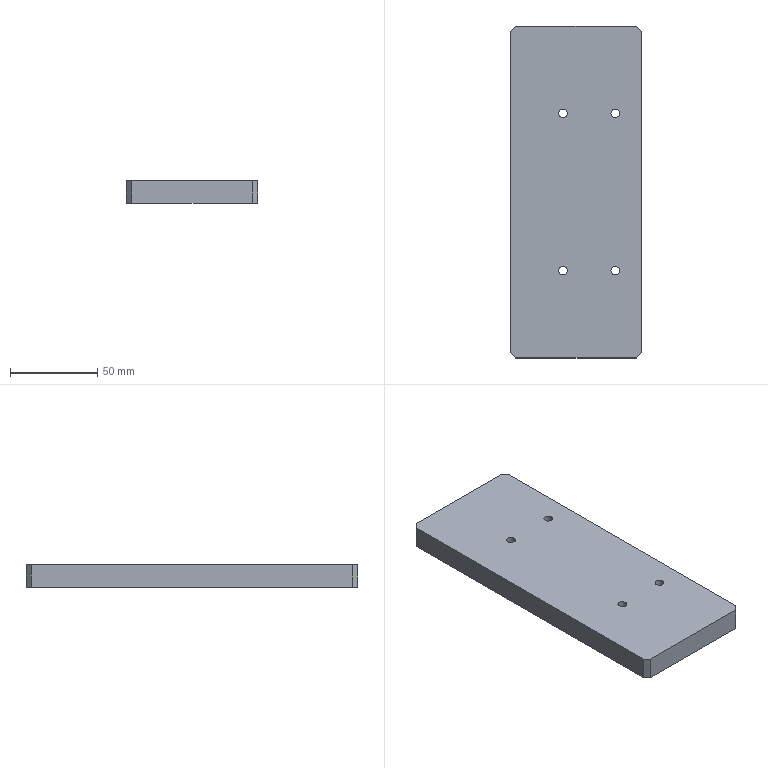Component | SolidWorks | STE21014.01-39-1 | 1 solid | 18 faces | box 75 x 190 x 13 mm | volume 183995 mm3 | plane 10 | cylinder 8 | commonest cylinder face diameters 5 x8 | material Q235
build123d program:
from build123d import *

# Parameters (mm, degrees)
SKETCH1_W           = 190
SKETCH1_H           = 75
BOSS_EXTRUDE1_DEPTH = 13
M6_TAPPED_HOLE1_D   = 5
CHAMFER1_SIZE       = 3


with BuildPart() as part:
    # Sketch1 → Boss-Extrude1 (new body)
    with BuildSketch(Plane(origin=(0, 0, 0), x_dir=(1, 0, 0), z_dir=(0, 1, 0))):
        Rectangle(SKETCH1_W, SKETCH1_H)
    extrude(amount=BOSS_EXTRUDE1_DEPTH)

    # M6 Tapped Hole1 (through all)
    with Locations(Plane(origin=(0, 13, 0), x_dir=(1, 0, 0), z_dir=(0, 1, 0))):
        with Locations((45, -7.5), (45, 22.5), (-45, -7.5), (-45, 22.5)):
            Hole(M6_TAPPED_HOLE1_D / 2)

    # Chamfer1
    chamfer1_edges = [part.edges().sort_by_distance(p)[0] for p in [
        (-95, 6.5, -37.5),
        (95, 6.5, -37.5),
        (95, 6.5, 37.5),
        (-95, 6.5, 37.5),
    ]]
    chamfer(chamfer1_edges, length=CHAMFER1_SIZE)


solid = part.part

# Placed as in the assembly
solid = solid.moved(Location((107.5, 80, -623), (90, -90, 0)))
STEP:
#1=COLOUR_RGB('',0.7922,0.8196,0.9333);
#2=FILL_AREA_STYLE_COLOUR('',#1);
#3=FILL_AREA_STYLE('',(#2));
#4=SURFACE_STYLE_FILL_AREA(#3);
#5=SURFACE_SIDE_STYLE('',(#4));
#6=SURFACE_STYLE_USAGE(.BOTH.,#5);
#7=PRESENTATION_STYLE_ASSIGNMENT((#6));
#8=CARTESIAN_POINT('',(4.035,4.921,-24.016));
#9=VERTEX_POINT('',#8);
#10=CARTESIAN_POINT('',(3.839,4.921,-24.016));
#11=VERTEX_POINT('',#10);
#12=CARTESIAN_POINT('',(3.937,4.921,-24.016));
#13=DIRECTION('',(-0.,-0.,-1.));
#14=DIRECTION('',(-1.,0.,0.));
#15=AXIS2_PLACEMENT_3D('',#12,#13,#14);
#16=CIRCLE('',#15,0.09843);
#17=EDGE_CURVE('',#9,#11,#16,.T.);
#18=ORIENTED_EDGE('',*,*,#17,.F.);
#19=CARTESIAN_POINT('',(4.035,4.921,-24.528));
#20=VERTEX_POINT('',#19);
#21=CARTESIAN_POINT('',(4.035,4.921,-24.528));
#22=DIRECTION('',(-0.,-0.,-1.));
#23=VECTOR('',#22,39.37);
#24=LINE('',#21,#23);
#25=EDGE_CURVE('',#9,#20,#24,.T.);
#26=ORIENTED_EDGE('',*,*,#25,.T.);
#27=CARTESIAN_POINT('',(3.839,4.921,-24.528));
#28=VERTEX_POINT('',#27);
#29=CARTESIAN_POINT('',(3.937,4.921,-24.528));
#30=DIRECTION('',(-0.,-0.,-1.));
#31=DIRECTION('',(-1.,0.,0.));
#32=AXIS2_PLACEMENT_3D('',#29,#30,#31);
#33=CIRCLE('',#32,0.09843);
#34=EDGE_CURVE('',#20,#28,#33,.T.);
#35=ORIENTED_EDGE('',*,*,#34,.T.);
#36=CARTESIAN_POINT('',(3.839,4.921,-24.528));
#37=DIRECTION('',(-0.,-0.,-1.));
#38=VECTOR('',#37,39.37);
#39=LINE('',#36,#38);
#40=EDGE_CURVE('',#11,#28,#39,.T.);
#41=ORIENTED_EDGE('',*,*,#40,.F.);
#42=EDGE_LOOP('',(#18,#26,#35,#41));
#43=FACE_OUTER_BOUND('',#42,.T.);
#44=CARTESIAN_POINT('',(3.937,4.921,-24.528));
#45=DIRECTION('',(-0.,-0.,-1.));
#46=DIRECTION('',(-1.,0.,0.));
#47=AXIS2_PLACEMENT_3D('',#44,#45,#46);
#48=CYLINDRICAL_SURFACE('',#47,0.09843);
#49=ADVANCED_FACE('',(#43),#48,.F.);
#50=CARTESIAN_POINT('',(5.217,4.921,-24.016));
#51=VERTEX_POINT('',#50);
#52=CARTESIAN_POINT('',(5.02,4.921,-24.016));
#53=VERTEX_POINT('',#52);
#54=CARTESIAN_POINT('',(5.118,4.921,-24.016));
#55=DIRECTION('',(-0.,-0.,-1.));
#56=DIRECTION('',(-1.,0.,0.));
#57=AXIS2_PLACEMENT_3D('',#54,#55,#56);
#58=CIRCLE('',#57,0.09843);
#59=EDGE_CURVE('',#51,#53,#58,.T.);
#60=ORIENTED_EDGE('',*,*,#59,.F.);
#61=CARTESIAN_POINT('',(5.217,4.921,-24.528));
#62=VERTEX_POINT('',#61);
#63=CARTESIAN_POINT('',(5.217,4.921,-24.528));
#64=DIRECTION('',(-0.,-0.,-1.));
#65=VECTOR('',#64,39.37);
#66=LINE('',#63,#65);
#67=EDGE_CURVE('',#51,#62,#66,.T.);
#68=ORIENTED_EDGE('',*,*,#67,.T.);
#69=CARTESIAN_POINT('',(5.02,4.921,-24.528));
#70=VERTEX_POINT('',#69);
#71=CARTESIAN_POINT('',(5.118,4.921,-24.528));
#72=DIRECTION('',(-0.,-0.,-1.));
#73=DIRECTION('',(-1.,0.,0.));
#74=AXIS2_PLACEMENT_3D('',#71,#72,#73);
#75=CIRCLE('',#74,0.09843);
#76=EDGE_CURVE('',#62,#70,#75,.T.);
#77=ORIENTED_EDGE('',*,*,#76,.T.);
#78=CARTESIAN_POINT('',(5.02,4.921,-24.528));
#79=DIRECTION('',(-0.,-0.,-1.));
#80=VECTOR('',#79,39.37);
#81=LINE('',#78,#80);
#82=EDGE_CURVE('',#53,#70,#81,.T.);
#83=ORIENTED_EDGE('',*,*,#82,.F.);
#84=EDGE_LOOP('',(#60,#68,#77,#83));
#85=FACE_OUTER_BOUND('',#84,.T.);
#86=CARTESIAN_POINT('',(5.118,4.921,-24.528));
#87=DIRECTION('',(-0.,-0.,-1.));
#88=DIRECTION('',(-1.,0.,0.));
#89=AXIS2_PLACEMENT_3D('',#86,#87,#88);
#90=CYLINDRICAL_SURFACE('',#89,0.09843);
#91=ADVANCED_FACE('',(#85),#90,.F.);
#92=CARTESIAN_POINT('',(4.035,1.378,-24.016));
#93=VERTEX_POINT('',#92);
#94=CARTESIAN_POINT('',(3.839,1.378,-24.016));
#95=VERTEX_POINT('',#94);
#96=CARTESIAN_POINT('',(3.937,1.378,-24.016));
#97=DIRECTION('',(-0.,-0.,-1.));
#98=DIRECTION('',(-1.,0.,0.));
#99=AXIS2_PLACEMENT_3D('',#96,#97,#98);
#100=CIRCLE('',#99,0.09843);
#101=EDGE_CURVE('',#93,#95,#100,.T.);
#102=ORIENTED_EDGE('',*,*,#101,.F.);
#103=CARTESIAN_POINT('',(4.035,1.378,-24.528));
#104=VERTEX_POINT('',#103);
#105=CARTESIAN_POINT('',(4.035,1.378,-24.528));
#106=DIRECTION('',(-0.,-0.,-1.));
#107=VECTOR('',#106,39.37);
#108=LINE('',#105,#107);
#109=EDGE_CURVE('',#93,#104,#108,.T.);
#110=ORIENTED_EDGE('',*,*,#109,.T.);
#111=CARTESIAN_POINT('',(3.839,1.378,-24.528));
#112=VERTEX_POINT('',#111);
#113=CARTESIAN_POINT('',(3.937,1.378,-24.528));
#114=DIRECTION('',(-0.,-0.,-1.));
#115=DIRECTION('',(-1.,0.,0.));
#116=AXIS2_PLACEMENT_3D('',#113,#114,#115);
#117=CIRCLE('',#116,0.09843);
#118=EDGE_CURVE('',#104,#112,#117,.T.);
#119=ORIENTED_EDGE('',*,*,#118,.T.);
#120=CARTESIAN_POINT('',(3.839,1.378,-24.528));
#121=DIRECTION('',(-0.,-0.,-1.));
#122=VECTOR('',#121,39.37);
#123=LINE('',#120,#122);
#124=EDGE_CURVE('',#95,#112,#123,.T.);
#125=ORIENTED_EDGE('',*,*,#124,.F.);
#126=EDGE_LOOP('',(#102,#110,#119,#125));
#127=FACE_OUTER_BOUND('',#126,.T.);
#128=CARTESIAN_POINT('',(3.937,1.378,-24.528));
#129=DIRECTION('',(-0.,-0.,-1.));
#130=DIRECTION('',(-1.,0.,0.));
#131=AXIS2_PLACEMENT_3D('',#128,#129,#130);
#132=CYLINDRICAL_SURFACE('',#131,0.09843);
#133=ADVANCED_FACE('',(#127),#132,.F.);
#134=CARTESIAN_POINT('',(5.217,1.378,-24.016));
#135=VERTEX_POINT('',#134);
#136=CARTESIAN_POINT('',(5.02,1.378,-24.016));
#137=VERTEX_POINT('',#136);
#138=CARTESIAN_POINT('',(5.118,1.378,-24.016));
#139=DIRECTION('',(-0.,-0.,-1.));
#140=DIRECTION('',(-1.,0.,0.));
#141=AXIS2_PLACEMENT_3D('',#138,#139,#140);
#142=CIRCLE('',#141,0.09843);
#143=EDGE_CURVE('',#135,#137,#142,.T.);
#144=ORIENTED_EDGE('',*,*,#143,.F.);
#145=CARTESIAN_POINT('',(5.217,1.378,-24.528));
#146=VERTEX_POINT('',#145);
#147=CARTESIAN_POINT('',(5.217,1.378,-24.528));
#148=DIRECTION('',(-0.,-0.,-1.));
#149=VECTOR('',#148,39.37);
#150=LINE('',#147,#149);
#151=EDGE_CURVE('',#135,#146,#150,.T.);
#152=ORIENTED_EDGE('',*,*,#151,.T.);
#153=CARTESIAN_POINT('',(5.02,1.378,-24.528));
#154=VERTEX_POINT('',#153);
#155=CARTESIAN_POINT('',(5.118,1.378,-24.528));
#156=DIRECTION('',(-0.,-0.,-1.));
#157=DIRECTION('',(-1.,0.,0.));
#158=AXIS2_PLACEMENT_3D('',#155,#156,#157);
#159=CIRCLE('',#158,0.09843);
#160=EDGE_CURVE('',#146,#154,#159,.T.);
#161=ORIENTED_EDGE('',*,*,#160,.T.);
#162=CARTESIAN_POINT('',(5.02,1.378,-24.528));
#163=DIRECTION('',(-0.,-0.,-1.));
#164=VECTOR('',#163,39.37);
#165=LINE('',#162,#164);
#166=EDGE_CURVE('',#137,#154,#165,.T.);
#167=ORIENTED_EDGE('',*,*,#166,.F.);
#168=EDGE_LOOP('',(#144,#152,#161,#167));
#169=FACE_OUTER_BOUND('',#168,.T.);
#170=CARTESIAN_POINT('',(5.118,1.378,-24.528));
#171=DIRECTION('',(-0.,-0.,-1.));
#172=DIRECTION('',(-1.,0.,0.));
#173=AXIS2_PLACEMENT_3D('',#170,#171,#172);
#174=CYLINDRICAL_SURFACE('',#173,0.09843);
#175=ADVANCED_FACE('',(#169),#174,.F.);
#176=CARTESIAN_POINT('',(5.591,-0.5906,-24.528));
#177=VERTEX_POINT('',#176);
#178=CARTESIAN_POINT('',(2.874,-0.5906,-24.528));
#179=VERTEX_POINT('',#178);
#180=CARTESIAN_POINT('',(2.756,-0.5906,-24.528));
#181=DIRECTION('',(-1.,-0.,0.));
#182=VECTOR('',#181,39.37);
#183=LINE('',#180,#182);
#184=EDGE_CURVE('',#177,#179,#183,.T.);
#185=ORIENTED_EDGE('',*,*,#184,.F.);
#186=CARTESIAN_POINT('',(5.591,-0.5906,-24.016));
#187=VERTEX_POINT('',#186);
#188=CARTESIAN_POINT('',(5.591,-0.5906,-24.528));
#189=DIRECTION('',(0.,0.,1.));
#190=VECTOR('',#189,39.37);
#191=LINE('',#188,#190);
#192=EDGE_CURVE('',#177,#187,#191,.T.);
#193=ORIENTED_EDGE('',*,*,#192,.T.);
#194=CARTESIAN_POINT('',(2.874,-0.5906,-24.016));
#195=VERTEX_POINT('',#194);
#196=CARTESIAN_POINT('',(2.756,-0.5906,-24.016));
#197=DIRECTION('',(-1.,-0.,0.));
#198=VECTOR('',#197,39.37);
#199=LINE('',#196,#198);
#200=EDGE_CURVE('',#187,#195,#199,.T.);
#201=ORIENTED_EDGE('',*,*,#200,.T.);
#202=CARTESIAN_POINT('',(2.874,-0.5906,-24.528));
#203=DIRECTION('',(-0.,-0.,-1.));
#204=VECTOR('',#203,39.37);
#205=LINE('',#202,#204);
#206=EDGE_CURVE('',#195,#179,#205,.T.);
#207=ORIENTED_EDGE('',*,*,#206,.T.);
#208=EDGE_LOOP('',(#185,#193,#201,#207));
#209=FACE_OUTER_BOUND('',#208,.T.);
#210=CARTESIAN_POINT('',(2.756,-0.5906,-24.528));
#211=DIRECTION('',(-0.,1.,-0.));
#212=DIRECTION('',(1.,0.,-0.));
#213=AXIS2_PLACEMENT_3D('',#210,#211,#212);
#214=PLANE('',#213);
#215=ADVANCED_FACE('',(#209),#214,.F.);
#216=CARTESIAN_POINT('',(2.756,-0.4724,-24.016));
#217=VERTEX_POINT('',#216);
#218=CARTESIAN_POINT('',(2.756,6.772,-24.016));
#219=VERTEX_POINT('',#218);
#220=CARTESIAN_POINT('',(2.756,6.89,-24.016));
#221=DIRECTION('',(0.,1.,-0.));
#222=VECTOR('',#221,39.37);
#223=LINE('',#220,#222);
#224=EDGE_CURVE('',#217,#219,#223,.T.);
#225=ORIENTED_EDGE('',*,*,#224,.T.);
#226=CARTESIAN_POINT('',(2.756,6.772,-24.528));
#227=VERTEX_POINT('',#226);
#228=CARTESIAN_POINT('',(2.756,6.772,-24.528));
#229=DIRECTION('',(-0.,-0.,-1.));
#230=VECTOR('',#229,39.37);
#231=LINE('',#228,#230);
#232=EDGE_CURVE('',#219,#227,#231,.T.);
#233=ORIENTED_EDGE('',*,*,#232,.T.);
#234=CARTESIAN_POINT('',(2.756,-0.4724,-24.528));
#235=VERTEX_POINT('',#234);
#236=CARTESIAN_POINT('',(2.756,6.89,-24.528));
#237=DIRECTION('',(0.,1.,-0.));
#238=VECTOR('',#237,39.37);
#239=LINE('',#236,#238);
#240=EDGE_CURVE('',#235,#227,#239,.T.);
#241=ORIENTED_EDGE('',*,*,#240,.F.);
#242=CARTESIAN_POINT('',(2.756,-0.4724,-24.528));
#243=DIRECTION('',(0.,0.,1.));
#244=VECTOR('',#243,39.37);
#245=LINE('',#242,#244);
#246=EDGE_CURVE('',#235,#217,#245,.T.);
#247=ORIENTED_EDGE('',*,*,#246,.T.);
#248=EDGE_LOOP('',(#225,#233,#241,#247));
#249=FACE_OUTER_BOUND('',#248,.T.);
#250=CARTESIAN_POINT('',(2.756,6.89,-24.528));
#251=DIRECTION('',(1.,-0.,-0.));
#252=DIRECTION('',(-0.,-1.,0.));
#253=AXIS2_PLACEMENT_3D('',#250,#251,#252);
#254=PLANE('',#253);
#255=ADVANCED_FACE('',(#249),#254,.F.);
#256=CARTESIAN_POINT('',(2.874,6.89,-24.528));
#257=VERTEX_POINT('',#256);
#258=CARTESIAN_POINT('',(5.591,6.89,-24.528));
#259=VERTEX_POINT('',#258);
#260=CARTESIAN_POINT('',(2.756,6.89,-24.528));
#261=DIRECTION('',(1.,0.,-0.));
#262=VECTOR('',#261,39.37);
#263=LINE('',#260,#262);
#264=EDGE_CURVE('',#257,#259,#263,.T.);
#265=ORIENTED_EDGE('',*,*,#264,.F.);
#266=CARTESIAN_POINT('',(2.874,6.89,-24.016));
#267=VERTEX_POINT('',#266);
#268=CARTESIAN_POINT('',(2.874,6.89,-24.528));
#269=DIRECTION('',(0.,0.,1.));
#270=VECTOR('',#269,39.37);
#271=LINE('',#268,#270);
#272=EDGE_CURVE('',#257,#267,#271,.T.);
#273=ORIENTED_EDGE('',*,*,#272,.T.);
#274=CARTESIAN_POINT('',(5.591,6.89,-24.016));
#275=VERTEX_POINT('',#274);
#276=CARTESIAN_POINT('',(2.756,6.89,-24.016));
#277=DIRECTION('',(1.,0.,-0.));
#278=VECTOR('',#277,39.37);
#279=LINE('',#276,#278);
#280=EDGE_CURVE('',#267,#275,#279,.T.);
#281=ORIENTED_EDGE('',*,*,#280,.T.);
#282=CARTESIAN_POINT('',(5.591,6.89,-24.528));
#283=DIRECTION('',(-0.,-0.,-1.));
#284=VECTOR('',#283,39.37);
#285=LINE('',#282,#284);
#286=EDGE_CURVE('',#275,#259,#285,.T.);
#287=ORIENTED_EDGE('',*,*,#286,.T.);
#288=EDGE_LOOP('',(#265,#273,#281,#287));
#289=FACE_OUTER_BOUND('',#288,.T.);
#290=CARTESIAN_POINT('',(2.756,6.89,-24.528));
#291=DIRECTION('',(0.,-1.,0.));
#292=DIRECTION('',(-1.,-0.,0.));
#293=AXIS2_PLACEMENT_3D('',#290,#291,#292);
#294=PLANE('',#293);
#295=ADVANCED_FACE('',(#289),#294,.F.);
#296=CARTESIAN_POINT('',(5.709,6.772,-24.528));
#297=VERTEX_POINT('',#296);
#298=CARTESIAN_POINT('',(5.709,-0.4724,-24.528));
#299=VERTEX_POINT('',#298);
#300=CARTESIAN_POINT('',(5.709,6.89,-24.528));
#301=DIRECTION('',(-0.,-1.,0.));
#302=VECTOR('',#301,39.37);
#303=LINE('',#300,#302);
#304=EDGE_CURVE('',#297,#299,#303,.T.);
#305=ORIENTED_EDGE('',*,*,#304,.F.);
#306=CARTESIAN_POINT('',(5.709,6.772,-24.016));
#307=VERTEX_POINT('',#306);
#308=CARTESIAN_POINT('',(5.709,6.772,-24.528));
#309=DIRECTION('',(0.,0.,1.));
#310=VECTOR('',#309,39.37);
#311=LINE('',#308,#310);
#312=EDGE_CURVE('',#297,#307,#311,.T.);
#313=ORIENTED_EDGE('',*,*,#312,.T.);
#314=CARTESIAN_POINT('',(5.709,-0.4724,-24.016));
#315=VERTEX_POINT('',#314);
#316=CARTESIAN_POINT('',(5.709,6.89,-24.016));
#317=DIRECTION('',(-0.,-1.,0.));
#318=VECTOR('',#317,39.37);
#319=LINE('',#316,#318);
#320=EDGE_CURVE('',#307,#315,#319,.T.);
#321=ORIENTED_EDGE('',*,*,#320,.T.);
#322=CARTESIAN_POINT('',(5.709,-0.4724,-24.528));
#323=DIRECTION('',(-0.,-0.,-1.));
#324=VECTOR('',#323,39.37);
#325=LINE('',#322,#324);
#326=EDGE_CURVE('',#315,#299,#325,.T.);
#327=ORIENTED_EDGE('',*,*,#326,.T.);
#328=EDGE_LOOP('',(#305,#313,#321,#327));
#329=FACE_OUTER_BOUND('',#328,.T.);
#330=CARTESIAN_POINT('',(5.709,6.89,-24.528));
#331=DIRECTION('',(-1.,0.,0.));
#332=DIRECTION('',(0.,1.,-0.));
#333=AXIS2_PLACEMENT_3D('',#330,#331,#332);
#334=PLANE('',#333);
#335=ADVANCED_FACE('',(#329),#334,.F.);
#336=CARTESIAN_POINT('',(3.937,4.921,-24.528));
#337=DIRECTION('',(-0.,-0.,-1.));
#338=DIRECTION('',(-1.,0.,0.));
#339=AXIS2_PLACEMENT_3D('',#336,#337,#338);
#340=CIRCLE('',#339,0.09843);
#341=EDGE_CURVE('',#28,#20,#340,.T.);
#342=ORIENTED_EDGE('',*,*,#341,.F.);
#343=ORIENTED_EDGE('',*,*,#34,.F.);
#344=EDGE_LOOP('',(#342,#343));
#345=FACE_BOUND('',#344,.T.);
#346=CARTESIAN_POINT('',(5.118,4.921,-24.528));
#347=DIRECTION('',(-0.,-0.,-1.));
#348=DIRECTION('',(-1.,0.,0.));
#349=AXIS2_PLACEMENT_3D('',#346,#347,#348);
#350=CIRCLE('',#349,0.09843);
#351=EDGE_CURVE('',#70,#62,#350,.T.);
#352=ORIENTED_EDGE('',*,*,#351,.F.);
#353=ORIENTED_EDGE('',*,*,#76,.F.);
#354=EDGE_LOOP('',(#352,#353));
#355=FACE_BOUND('',#354,.T.);
#356=CARTESIAN_POINT('',(3.937,1.378,-24.528));
#357=DIRECTION('',(-0.,-0.,-1.));
#358=DIRECTION('',(-1.,0.,0.));
#359=AXIS2_PLACEMENT_3D('',#356,#357,#358);
#360=CIRCLE('',#359,0.09843);
#361=EDGE_CURVE('',#112,#104,#360,.T.);
#362=ORIENTED_EDGE('',*,*,#361,.F.);
#363=ORIENTED_EDGE('',*,*,#118,.F.);
#364=EDGE_LOOP('',(#362,#363));
#365=FACE_BOUND('',#364,.T.);
#366=CARTESIAN_POINT('',(5.118,1.378,-24.528));
#367=DIRECTION('',(-0.,-0.,-1.));
#368=DIRECTION('',(-1.,0.,0.));
#369=AXIS2_PLACEMENT_3D('',#366,#367,#368);
#370=CIRCLE('',#369,0.09843);
#371=EDGE_CURVE('',#154,#146,#370,.T.);
#372=ORIENTED_EDGE('',*,*,#371,.F.);
#373=ORIENTED_EDGE('',*,*,#160,.F.);
#374=EDGE_LOOP('',(#372,#373));
#375=FACE_BOUND('',#374,.T.);
#376=ORIENTED_EDGE('',*,*,#240,.T.);
#377=CARTESIAN_POINT('',(1.683,5.699,-24.528));
#378=DIRECTION('',(0.7071,0.7071,-0.));
#379=VECTOR('',#378,39.37);
#380=LINE('',#377,#379);
#381=EDGE_CURVE('',#227,#257,#380,.T.);
#382=ORIENTED_EDGE('',*,*,#381,.T.);
#383=ORIENTED_EDGE('',*,*,#264,.T.);
#384=CARTESIAN_POINT('',(6.781,5.699,-24.528));
#385=DIRECTION('',(0.7071,-0.7071,0.));
#386=VECTOR('',#385,39.37);
#387=LINE('',#384,#386);
#388=EDGE_CURVE('',#259,#297,#387,.T.);
#389=ORIENTED_EDGE('',*,*,#388,.T.);
#390=ORIENTED_EDGE('',*,*,#304,.T.);
#391=CARTESIAN_POINT('',(6.781,0.6004,-24.528));
#392=DIRECTION('',(-0.7071,-0.7071,0.));
#393=VECTOR('',#392,39.37);
#394=LINE('',#391,#393);
#395=EDGE_CURVE('',#299,#177,#394,.T.);
#396=ORIENTED_EDGE('',*,*,#395,.T.);
#397=ORIENTED_EDGE('',*,*,#184,.T.);
#398=CARTESIAN_POINT('',(1.683,0.6004,-24.528));
#399=DIRECTION('',(-0.7071,0.7071,-0.));
#400=VECTOR('',#399,39.37);
#401=LINE('',#398,#400);
#402=EDGE_CURVE('',#179,#235,#401,.T.);
#403=ORIENTED_EDGE('',*,*,#402,.T.);
#404=EDGE_LOOP('',(#376,#382,#383,#389,#390,#396,#397,#403));
#405=FACE_OUTER_BOUND('',#404,.T.);
#406=CARTESIAN_POINT('',(4.232,3.15,-24.528));
#407=DIRECTION('',(-0.,-0.,-1.));
#408=DIRECTION('',(-1.,-0.,0.));
#409=AXIS2_PLACEMENT_3D('',#406,#407,#408);
#410=PLANE('',#409);
#411=ADVANCED_FACE('',(#345,#355,#365,#375,#405),#410,.T.);
#412=CARTESIAN_POINT('',(3.937,4.921,-24.016));
#413=DIRECTION('',(-0.,-0.,-1.));
#414=DIRECTION('',(-1.,0.,0.));
#415=AXIS2_PLACEMENT_3D('',#412,#413,#414);
#416=CIRCLE('',#415,0.09843);
#417=EDGE_CURVE('',#11,#9,#416,.T.);
#418=ORIENTED_EDGE('',*,*,#417,.T.);
#419=ORIENTED_EDGE('',*,*,#17,.T.);
#420=EDGE_LOOP('',(#418,#419));
#421=FACE_BOUND('',#420,.T.);
#422=CARTESIAN_POINT('',(5.118,4.921,-24.016));
#423=DIRECTION('',(-0.,-0.,-1.));
#424=DIRECTION('',(-1.,0.,0.));
#425=AXIS2_PLACEMENT_3D('',#422,#423,#424);
#426=CIRCLE('',#425,0.09843);
#427=EDGE_CURVE('',#53,#51,#426,.T.);
#428=ORIENTED_EDGE('',*,*,#427,.T.);
#429=ORIENTED_EDGE('',*,*,#59,.T.);
#430=EDGE_LOOP('',(#428,#429));
#431=FACE_BOUND('',#430,.T.);
#432=CARTESIAN_POINT('',(3.937,1.378,-24.016));
#433=DIRECTION('',(-0.,-0.,-1.));
#434=DIRECTION('',(-1.,0.,0.));
#435=AXIS2_PLACEMENT_3D('',#432,#433,#434);
#436=CIRCLE('',#435,0.09843);
#437=EDGE_CURVE('',#95,#93,#436,.T.);
#438=ORIENTED_EDGE('',*,*,#437,.T.);
#439=ORIENTED_EDGE('',*,*,#101,.T.);
#440=EDGE_LOOP('',(#438,#439));
#441=FACE_BOUND('',#440,.T.);
#442=CARTESIAN_POINT('',(5.118,1.378,-24.016));
#443=DIRECTION('',(-0.,-0.,-1.));
#444=DIRECTION('',(-1.,0.,0.));
#445=AXIS2_PLACEMENT_3D('',#442,#443,#444);
#446=CIRCLE('',#445,0.09843);
#447=EDGE_CURVE('',#137,#135,#446,.T.);
#448=ORIENTED_EDGE('',*,*,#447,.T.);
#449=ORIENTED_EDGE('',*,*,#143,.T.);
#450=EDGE_LOOP('',(#448,#449));
#451=FACE_BOUND('',#450,.T.);
#452=ORIENTED_EDGE('',*,*,#280,.F.);
#453=CARTESIAN_POINT('',(2.874,6.89,-24.016));
#454=DIRECTION('',(-0.7071,-0.7071,0.));
#455=VECTOR('',#454,39.37);
#456=LINE('',#453,#455);
#457=EDGE_CURVE('',#267,#219,#456,.T.);
#458=ORIENTED_EDGE('',*,*,#457,.T.);
#459=ORIENTED_EDGE('',*,*,#224,.F.);
#460=CARTESIAN_POINT('',(2.756,-0.4724,-24.016));
#461=DIRECTION('',(0.7071,-0.7071,0.));
#462=VECTOR('',#461,39.37);
#463=LINE('',#460,#462);
#464=EDGE_CURVE('',#217,#195,#463,.T.);
#465=ORIENTED_EDGE('',*,*,#464,.T.);
#466=ORIENTED_EDGE('',*,*,#200,.F.);
#467=CARTESIAN_POINT('',(5.591,-0.5906,-24.016));
#468=DIRECTION('',(0.7071,0.7071,-0.));
#469=VECTOR('',#468,39.37);
#470=LINE('',#467,#469);
#471=EDGE_CURVE('',#187,#315,#470,.T.);
#472=ORIENTED_EDGE('',*,*,#471,.T.);
#473=ORIENTED_EDGE('',*,*,#320,.F.);
#474=CARTESIAN_POINT('',(5.709,6.772,-24.016));
#475=DIRECTION('',(-0.7071,0.7071,-0.));
#476=VECTOR('',#475,39.37);
#477=LINE('',#474,#476);
#478=EDGE_CURVE('',#307,#275,#477,.T.);
#479=ORIENTED_EDGE('',*,*,#478,.T.);
#480=EDGE_LOOP('',(#452,#458,#459,#465,#466,#472,#473,#479));
#481=FACE_OUTER_BOUND('',#480,.T.);
#482=CARTESIAN_POINT('',(4.232,3.15,-24.016));
#483=DIRECTION('',(-0.,-0.,-1.));
#484=DIRECTION('',(-1.,-0.,0.));
#485=AXIS2_PLACEMENT_3D('',#482,#483,#484);
#486=PLANE('',#485);
#487=ADVANCED_FACE('',(#421,#431,#441,#451,#481),#486,.F.);
#488=ORIENTED_EDGE('',*,*,#151,.F.);
#489=ORIENTED_EDGE('',*,*,#447,.F.);
#490=ORIENTED_EDGE('',*,*,#166,.T.);
#491=ORIENTED_EDGE('',*,*,#371,.T.);
#492=EDGE_LOOP('',(#488,#489,#490,#491));
#493=FACE_OUTER_BOUND('',#492,.T.);
#494=CARTESIAN_POINT('',(5.118,1.378,-24.528));
#495=DIRECTION('',(-0.,-0.,-1.));
#496=DIRECTION('',(-1.,0.,0.));
#497=AXIS2_PLACEMENT_3D('',#494,#495,#496);
#498=CYLINDRICAL_SURFACE('',#497,0.09843);
#499=ADVANCED_FACE('',(#493),#498,.F.);
#500=ORIENTED_EDGE('',*,*,#109,.F.);
#501=ORIENTED_EDGE('',*,*,#437,.F.);
#502=ORIENTED_EDGE('',*,*,#124,.T.);
#503=ORIENTED_EDGE('',*,*,#361,.T.);
#504=EDGE_LOOP('',(#500,#501,#502,#503));
#505=FACE_OUTER_BOUND('',#504,.T.);
#506=CARTESIAN_POINT('',(3.937,1.378,-24.528));
#507=DIRECTION('',(-0.,-0.,-1.));
#508=DIRECTION('',(-1.,0.,0.));
#509=AXIS2_PLACEMENT_3D('',#506,#507,#508);
#510=CYLINDRICAL_SURFACE('',#509,0.09843);
#511=ADVANCED_FACE('',(#505),#510,.F.);
#512=ORIENTED_EDGE('',*,*,#67,.F.);
#513=ORIENTED_EDGE('',*,*,#427,.F.);
#514=ORIENTED_EDGE('',*,*,#82,.T.);
#515=ORIENTED_EDGE('',*,*,#351,.T.);
#516=EDGE_LOOP('',(#512,#513,#514,#515));
#517=FACE_OUTER_BOUND('',#516,.T.);
#518=CARTESIAN_POINT('',(5.118,4.921,-24.528));
#519=DIRECTION('',(-0.,-0.,-1.));
#520=DIRECTION('',(-1.,0.,0.));
#521=AXIS2_PLACEMENT_3D('',#518,#519,#520);
#522=CYLINDRICAL_SURFACE('',#521,0.09843);
#523=ADVANCED_FACE('',(#517),#522,.F.);
#524=ORIENTED_EDGE('',*,*,#25,.F.);
#525=ORIENTED_EDGE('',*,*,#417,.F.);
#526=ORIENTED_EDGE('',*,*,#40,.T.);
#527=ORIENTED_EDGE('',*,*,#341,.T.);
#528=EDGE_LOOP('',(#524,#525,#526,#527));
#529=FACE_OUTER_BOUND('',#528,.T.);
#530=CARTESIAN_POINT('',(3.937,4.921,-24.528));
#531=DIRECTION('',(-0.,-0.,-1.));
#532=DIRECTION('',(-1.,0.,0.));
#533=AXIS2_PLACEMENT_3D('',#530,#531,#532);
#534=CYLINDRICAL_SURFACE('',#533,0.09843);
#535=ADVANCED_FACE('',(#529),#534,.F.);
#536=ORIENTED_EDGE('',*,*,#381,.F.);
#537=ORIENTED_EDGE('',*,*,#232,.F.);
#538=ORIENTED_EDGE('',*,*,#457,.F.);
#539=ORIENTED_EDGE('',*,*,#272,.F.);
#540=EDGE_LOOP('',(#536,#537,#538,#539));
#541=FACE_OUTER_BOUND('',#540,.T.);
#542=CARTESIAN_POINT('',(2.874,6.89,-24.528));
#543=DIRECTION('',(0.7071,-0.7071,0.));
#544=DIRECTION('',(0.,0.,1.));
#545=AXIS2_PLACEMENT_3D('',#542,#543,#544);
#546=PLANE('',#545);
#547=ADVANCED_FACE('',(#541),#546,.F.);
#548=ORIENTED_EDGE('',*,*,#388,.F.);
#549=ORIENTED_EDGE('',*,*,#286,.F.);
#550=ORIENTED_EDGE('',*,*,#478,.F.);
#551=ORIENTED_EDGE('',*,*,#312,.F.);
#552=EDGE_LOOP('',(#548,#549,#550,#551));
#553=FACE_OUTER_BOUND('',#552,.T.);
#554=CARTESIAN_POINT('',(5.709,6.772,-24.528));
#555=DIRECTION('',(-0.7071,-0.7071,0.));
#556=DIRECTION('',(0.,0.,1.));
#557=AXIS2_PLACEMENT_3D('',#554,#555,#556);
#558=PLANE('',#557);
#559=ADVANCED_FACE('',(#553),#558,.F.);
#560=ORIENTED_EDGE('',*,*,#395,.F.);
#561=ORIENTED_EDGE('',*,*,#326,.F.);
#562=ORIENTED_EDGE('',*,*,#471,.F.);
#563=ORIENTED_EDGE('',*,*,#192,.F.);
#564=EDGE_LOOP('',(#560,#561,#562,#563));
#565=FACE_OUTER_BOUND('',#564,.T.);
#566=CARTESIAN_POINT('',(5.591,-0.5906,-24.528));
#567=DIRECTION('',(-0.7071,0.7071,-0.));
#568=DIRECTION('',(0.,0.,1.));
#569=AXIS2_PLACEMENT_3D('',#566,#567,#568);
#570=PLANE('',#569);
#571=ADVANCED_FACE('',(#565),#570,.F.);
#572=ORIENTED_EDGE('',*,*,#402,.F.);
#573=ORIENTED_EDGE('',*,*,#206,.F.);
#574=ORIENTED_EDGE('',*,*,#464,.F.);
#575=ORIENTED_EDGE('',*,*,#246,.F.);
#576=EDGE_LOOP('',(#572,#573,#574,#575));
#577=FACE_OUTER_BOUND('',#576,.T.);
#578=CARTESIAN_POINT('',(2.756,-0.4724,-24.528));
#579=DIRECTION('',(0.7071,0.7071,-0.));
#580=DIRECTION('',(0.,0.,1.));
#581=AXIS2_PLACEMENT_3D('',#578,#579,#580);
#582=PLANE('',#581);
#583=ADVANCED_FACE('',(#577),#582,.F.);
#584=CLOSED_SHELL('',(#49,#91,#133,#175,#215,#255,#295,#335,#411,#487,#499,#511,#523,#535,#547,#559,#571,#583));
#585=MANIFOLD_SOLID_BREP('',#584);
#586=STYLED_ITEM('',(#7),#585);
#587=(LENGTH_UNIT()NAMED_UNIT(*)SI_UNIT($,.METRE.));
#588=LENGTH_MEASURE_WITH_UNIT(LENGTH_MEASURE(0.0254),#587);
#589=DIMENSIONAL_EXPONENTS(1.,0.,0.,0.,0.,0.,0.);
#590=(CONVERSION_BASED_UNIT('',#588)LENGTH_UNIT()NAMED_UNIT(#589));
#591=UNCERTAINTY_MEASURE_WITH_UNIT(LENGTH_MEASURE(0.00001),#590,'','');
#592=(NAMED_UNIT(*)PLANE_ANGLE_UNIT()SI_UNIT($,.RADIAN.));
#593=(NAMED_UNIT(*)SI_UNIT($,.STERADIAN.)SOLID_ANGLE_UNIT());
#594=(GEOMETRIC_REPRESENTATION_CONTEXT(3)GLOBAL_UNCERTAINTY_ASSIGNED_CONTEXT((#591))GLOBAL_UNIT_ASSIGNED_CONTEXT((#590,#592,#593))REPRESENTATION_CONTEXT('',''));
#595=MECHANICAL_DESIGN_GEOMETRIC_PRESENTATION_REPRESENTATION('',(#586),#594);
#596=CARTESIAN_POINT('',(0.,0.,0.));
#597=DIRECTION('',(0.,0.,1.));
#598=DIRECTION('',(1.,0.,0.));
#599=AXIS2_PLACEMENT_3D('',#596,#597,#598);
#600=(LENGTH_UNIT()NAMED_UNIT(*)SI_UNIT($,.METRE.));
#601=LENGTH_MEASURE_WITH_UNIT(LENGTH_MEASURE(0.0254),#600);
#602=DIMENSIONAL_EXPONENTS(1.,0.,0.,0.,0.,0.,0.);
#603=(CONVERSION_BASED_UNIT('',#601)LENGTH_UNIT()NAMED_UNIT(#602));
#604=UNCERTAINTY_MEASURE_WITH_UNIT(LENGTH_MEASURE(0.00001),#603,'','');
#605=(NAMED_UNIT(*)PLANE_ANGLE_UNIT()SI_UNIT($,.RADIAN.));
#606=(NAMED_UNIT(*)SI_UNIT($,.STERADIAN.)SOLID_ANGLE_UNIT());
#607=(GEOMETRIC_REPRESENTATION_CONTEXT(3)GLOBAL_UNCERTAINTY_ASSIGNED_CONTEXT((#604))GLOBAL_UNIT_ASSIGNED_CONTEXT((#603,#605,#606))REPRESENTATION_CONTEXT('',''));
#608=ADVANCED_BREP_SHAPE_REPRESENTATION('',(#585,#599),#607);
#609=PRESENTATION_LAYER_ASSIGNMENT('','',(#586));